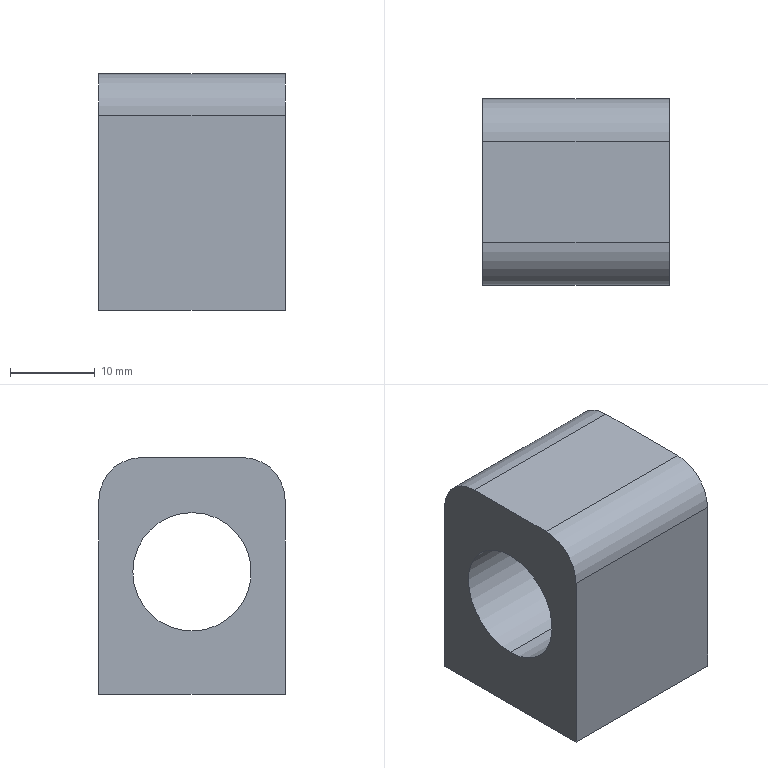CAM job | Mastercam | mm | 9 operations | part box 22 x 22 x 28
1. Facing | 24 - 100 平铣刀
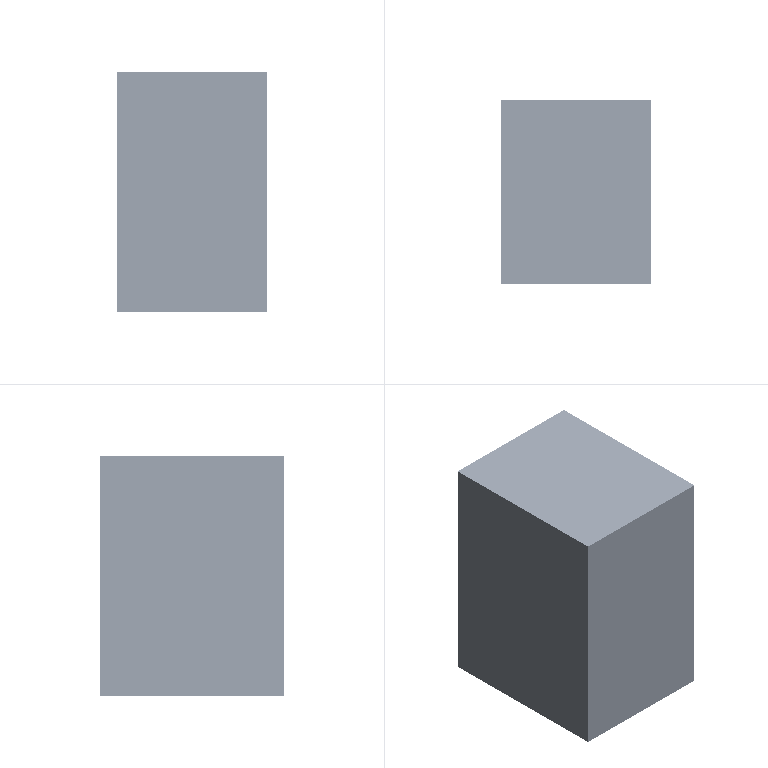2. Contour (Ramp) | 12 - 12 平铣刀
3. Contour (2D) | 12 - 12 平铣刀
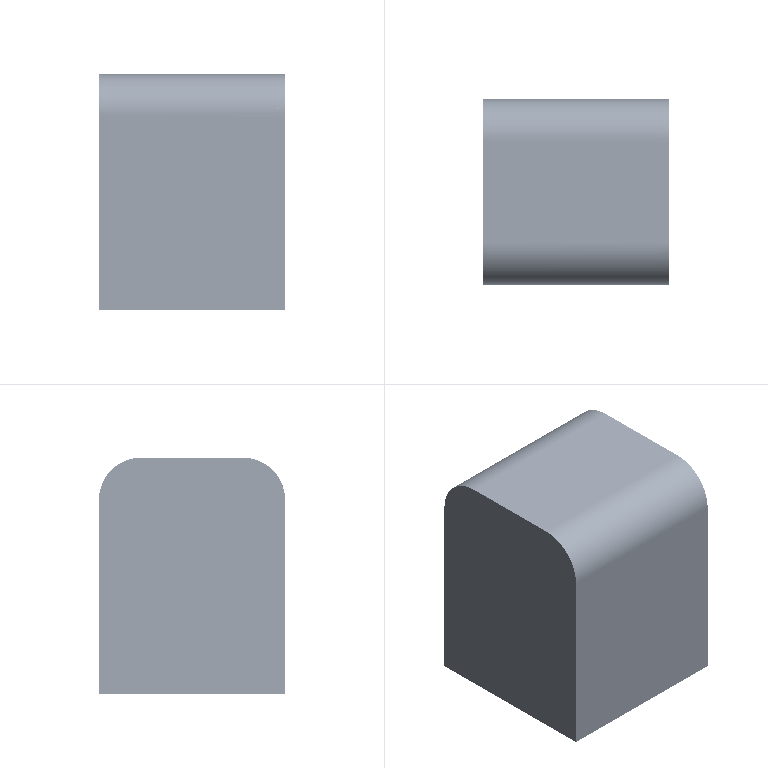4. Contour (Ramp) | 6 - 6 平铣刀
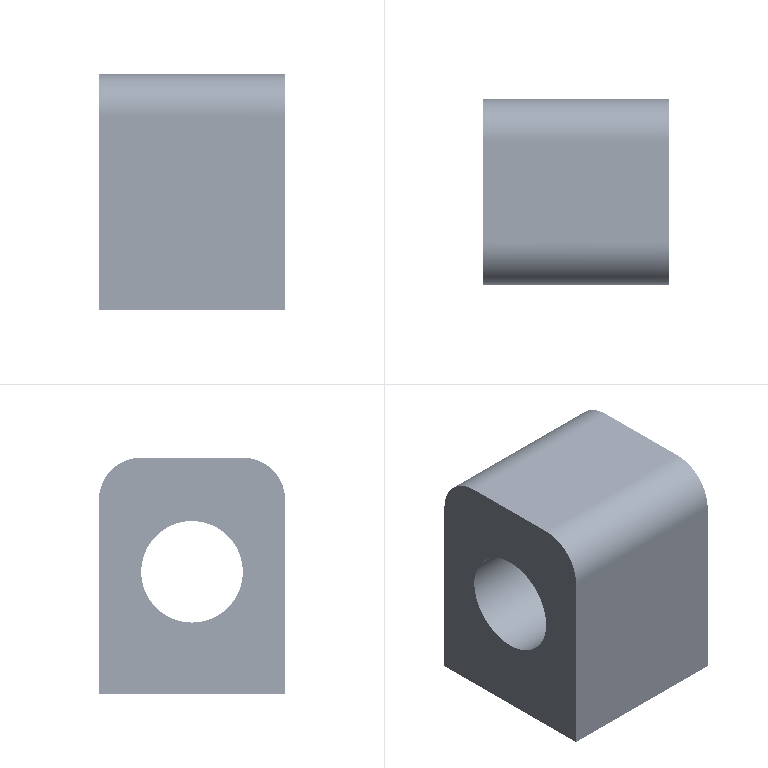5. Contour (Ramp) | 6 - 6 平铣刀
6. Contour (2D chamfer) | 7 - 4 倒角刀
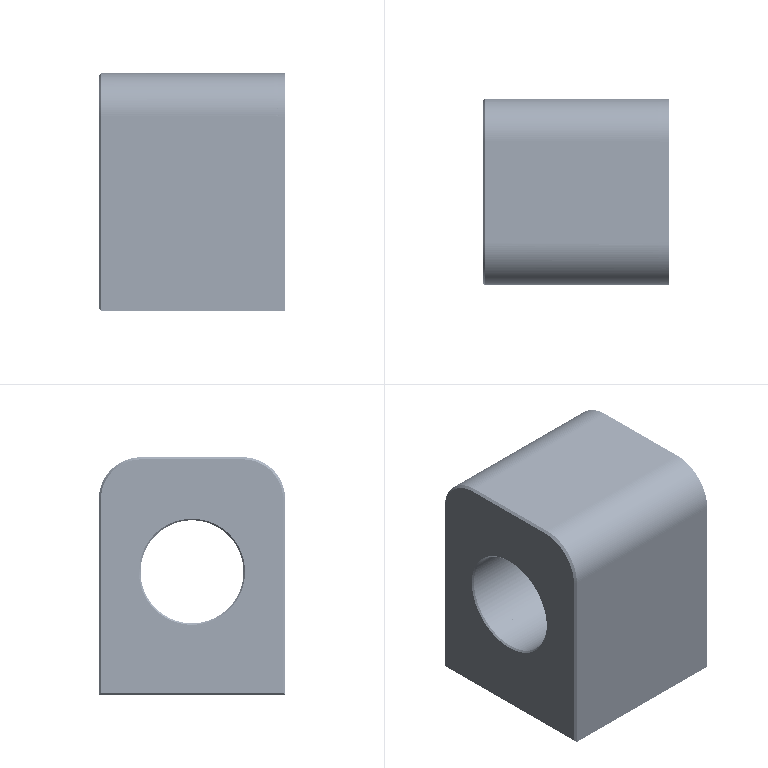7. Facing | 24 - 100 平铣刀
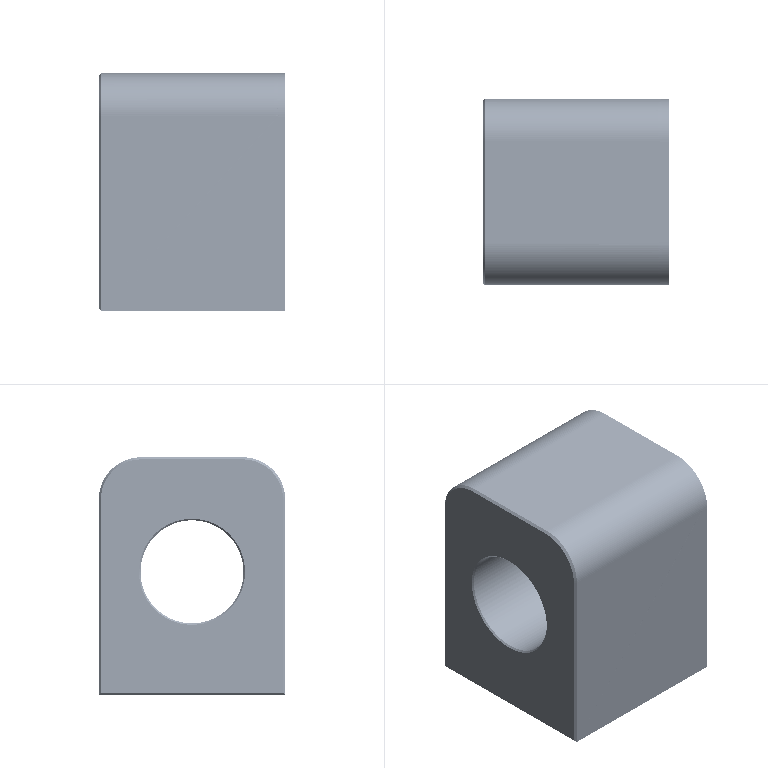8. Contour (2D chamfer) | 7 - 4 倒角刀
9. Drill/Counterbore | 7 - 4 倒角刀